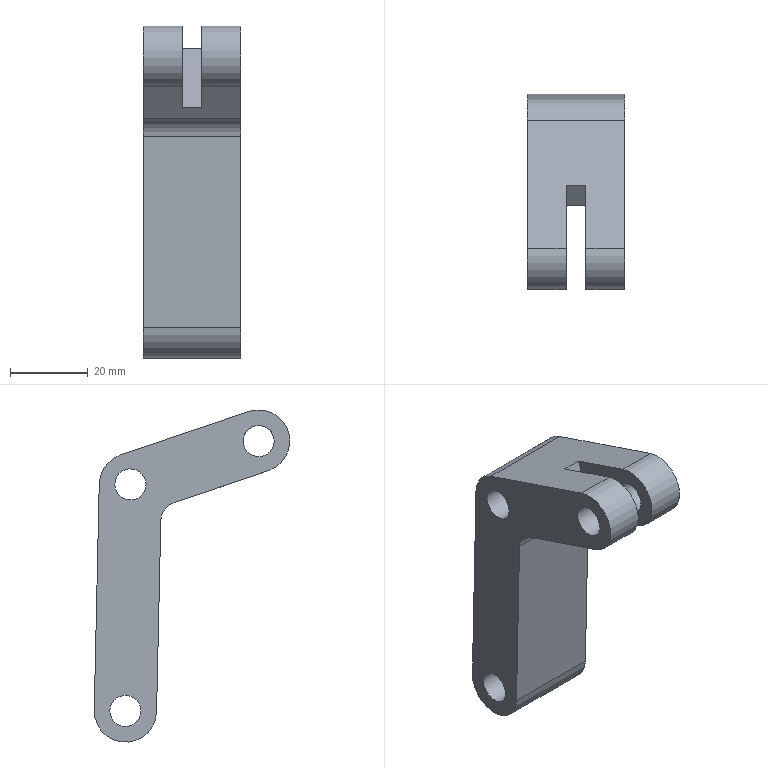Component | NX | JAWLINK | 1 solid | 18 faces | volume 36698 mm3 | plane 9 | cylinder 9 | commonest cylinder face diameters 8 x4 16 x4 10 x1